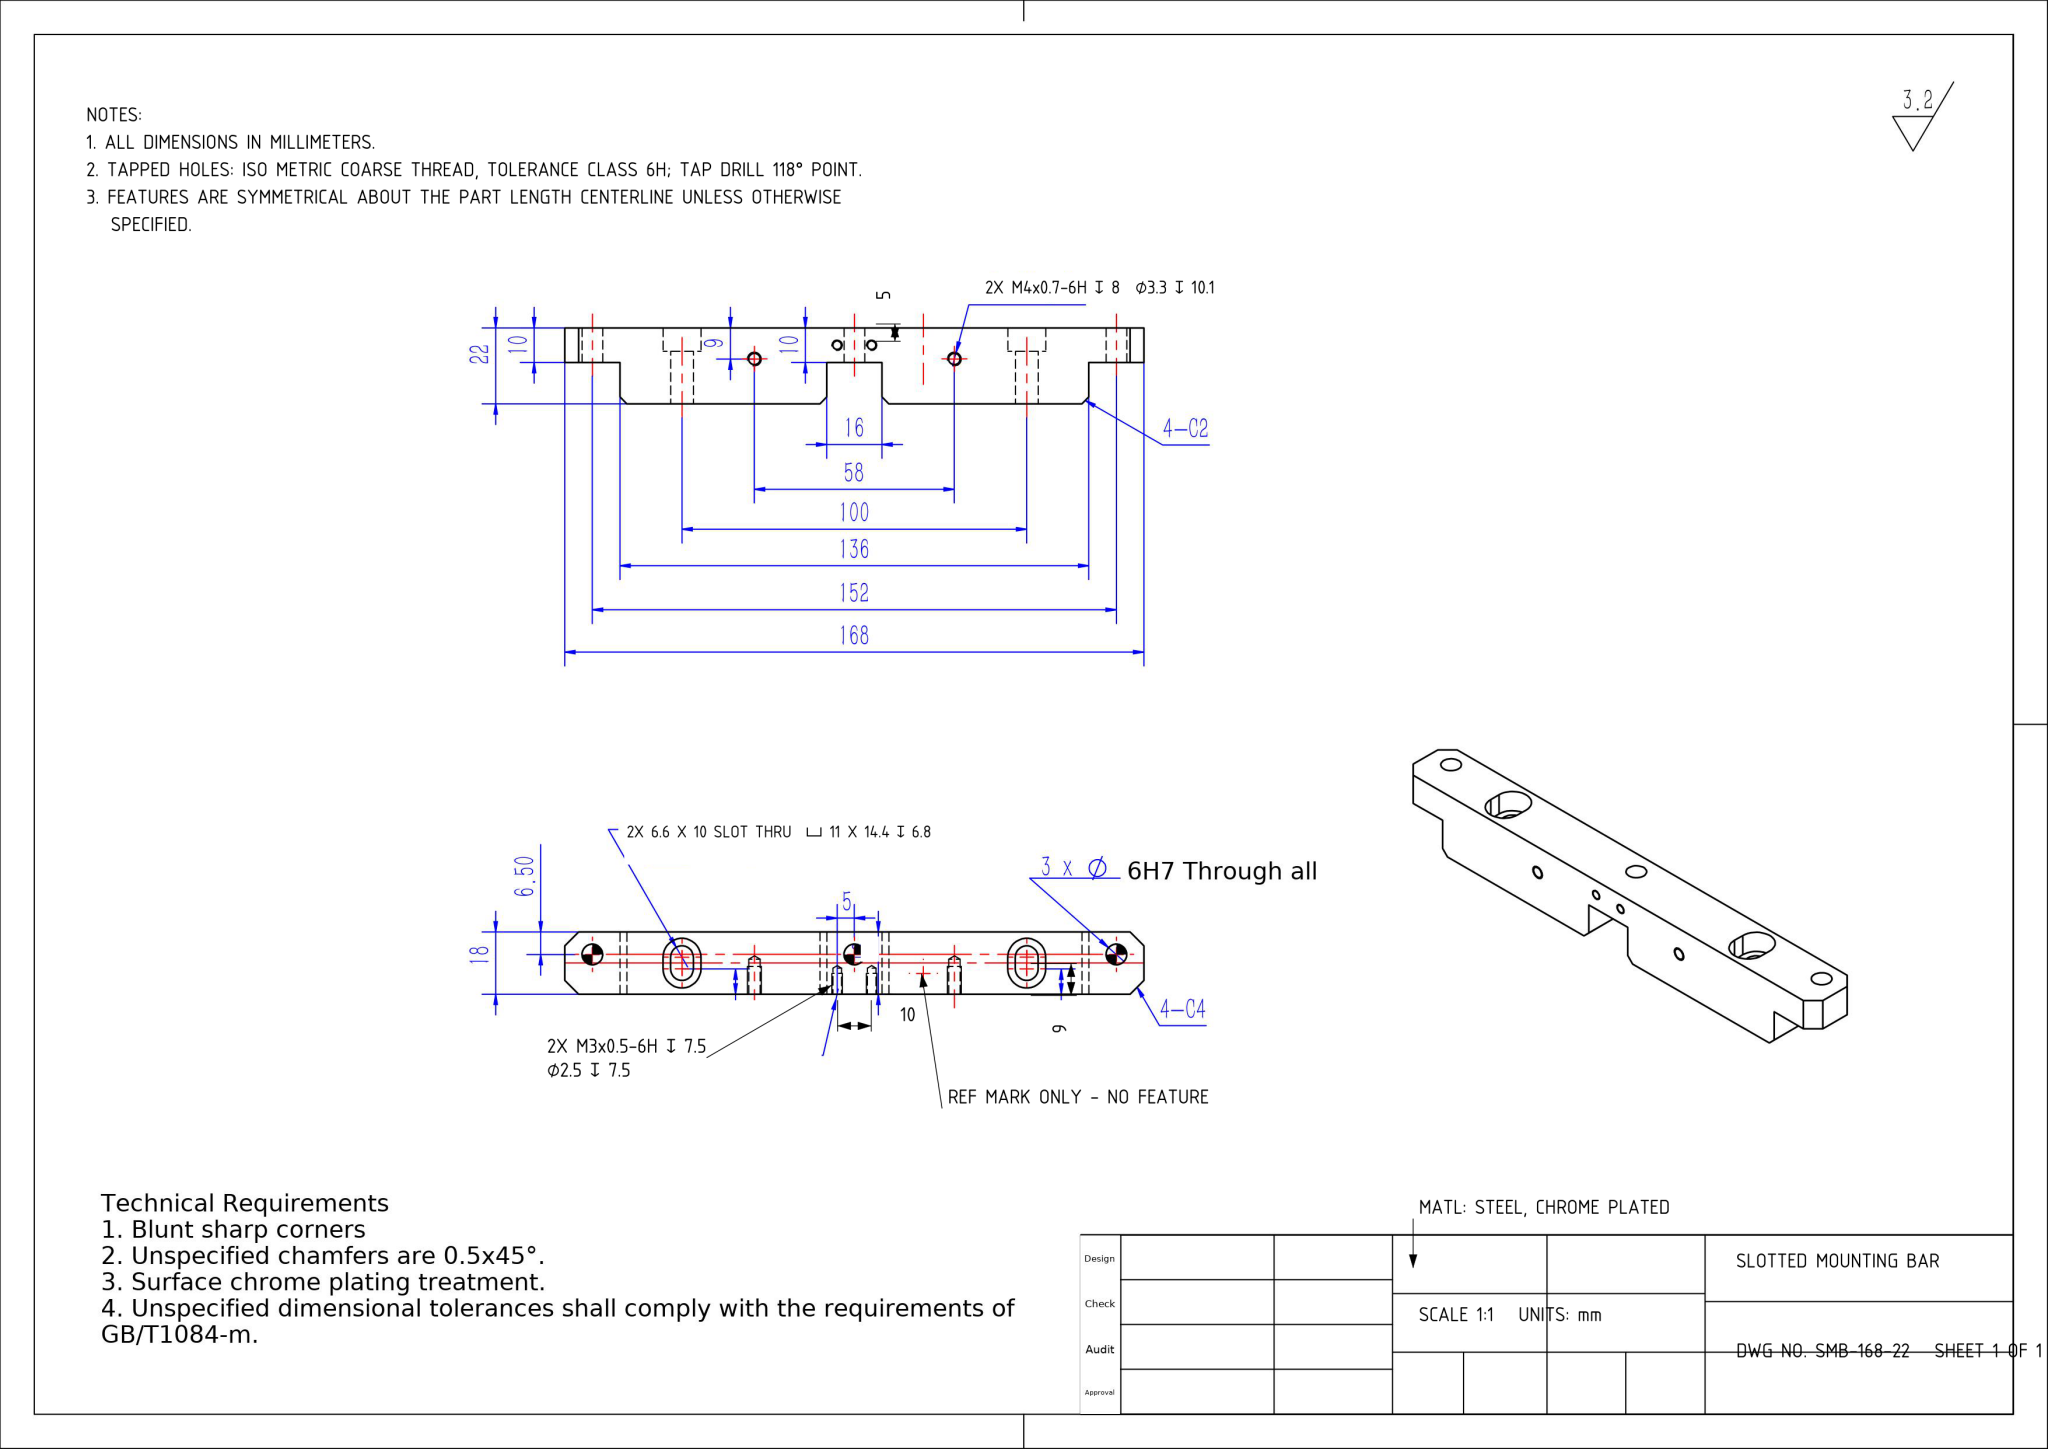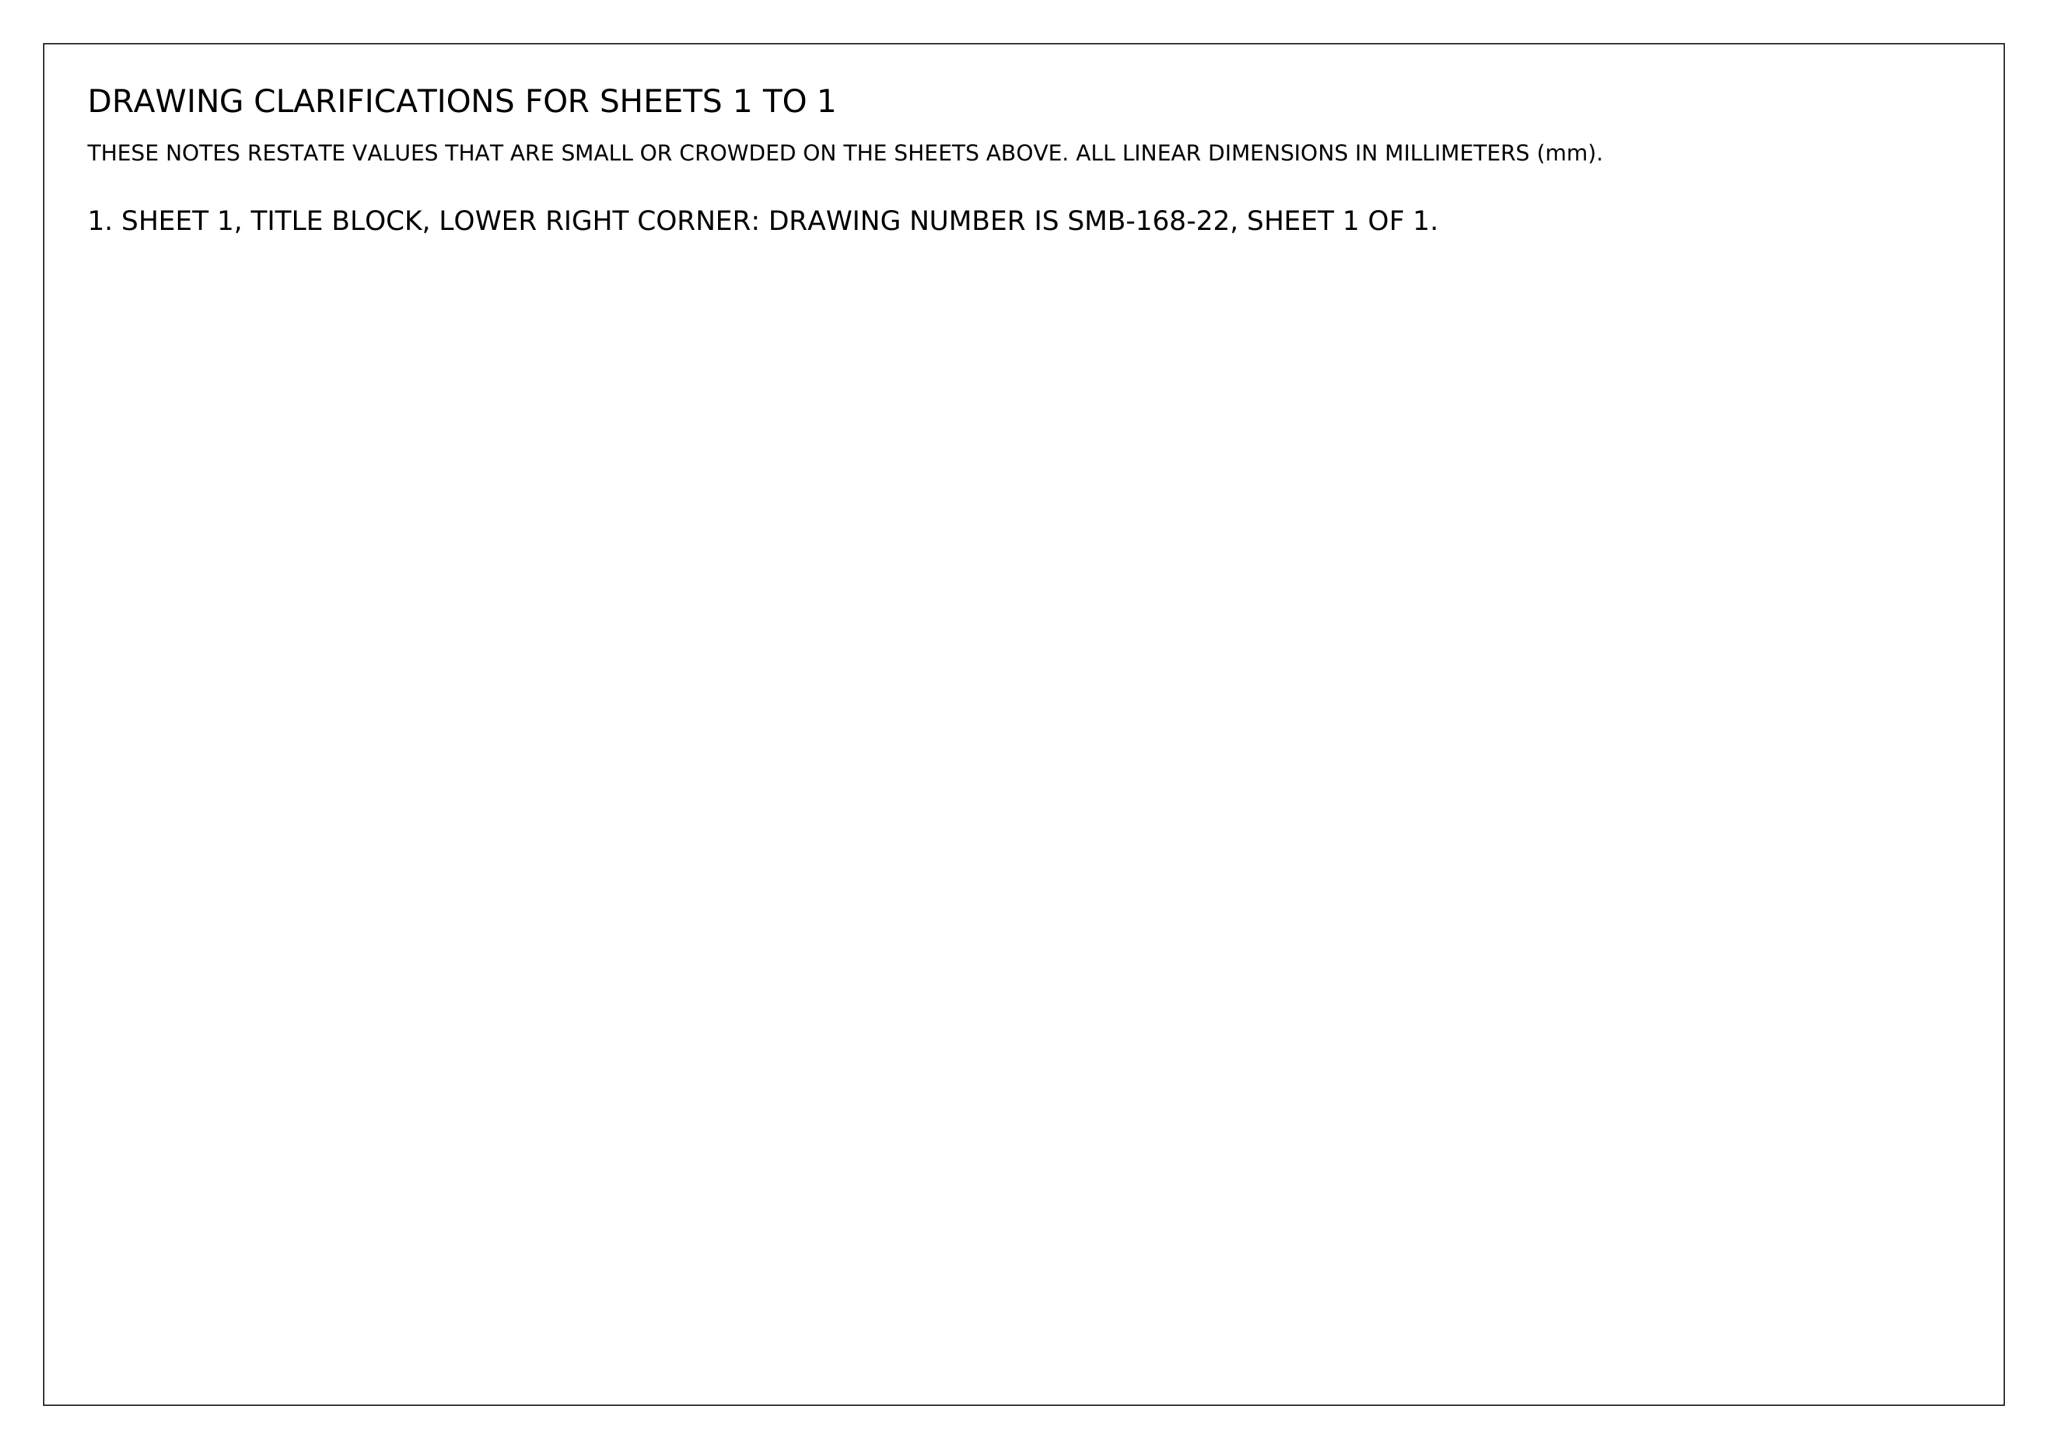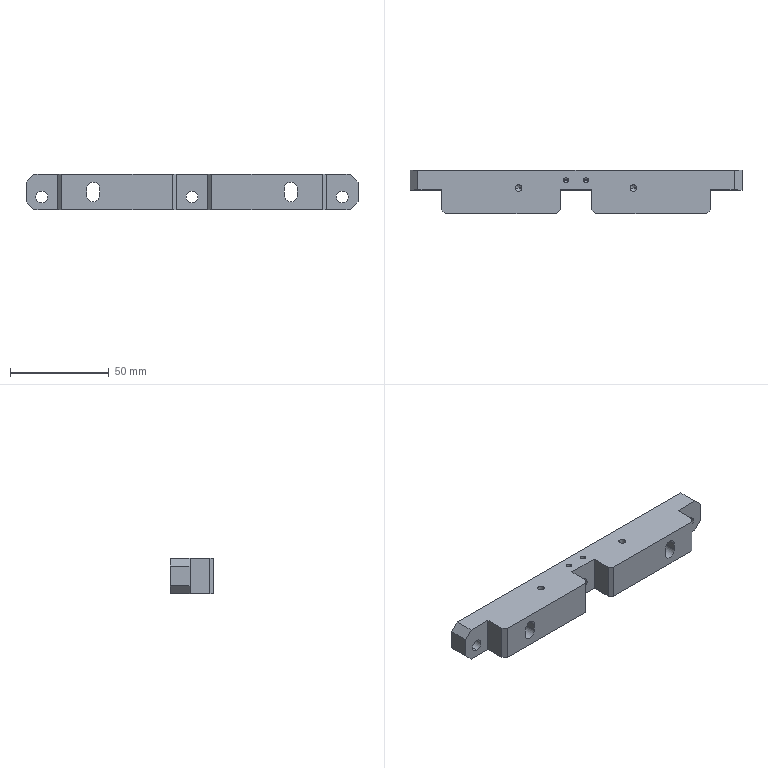Part | NX | mm | 1 solid | 66 faces | box 168 x 22 x 18 mm | volume 51070 mm3 | plane 32 | cylinder 26 | cone 8 | commonest cylinder face diameters 11 x6 6.6 x6 6 x6 3.3 x4 2.5 x4